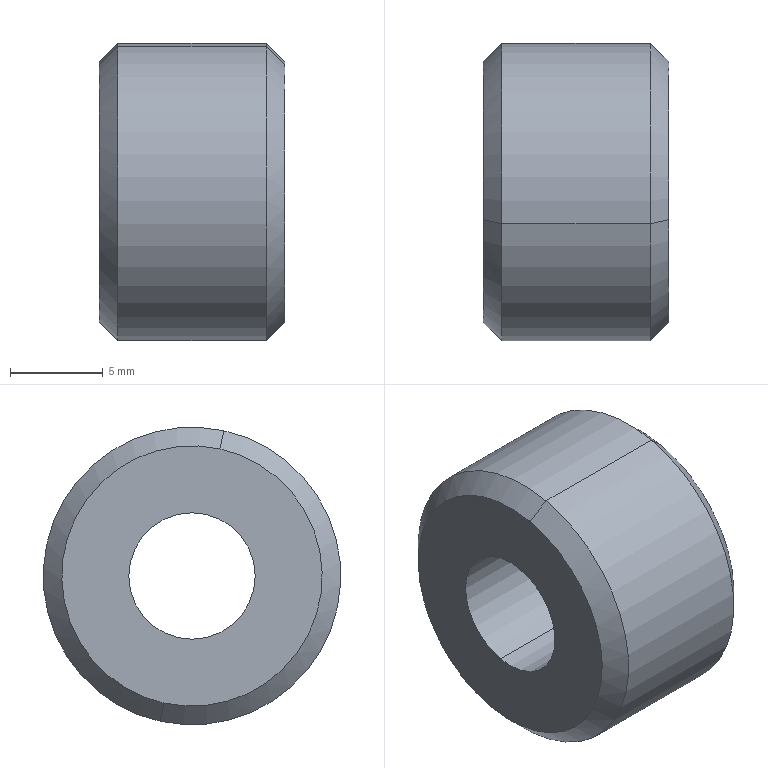Component | SolidWorks | 17SmallKnurledNut-1 | 1 solid | 12 faces | box 10 x 16 x 16 mm | volume 1595 mm3 | cone 6 | cylinder 4 | plane 2 | commonest cylinder face diameters 6.8 x2 16 x2
build123d program:
from build123d import *

# Parameters (mm, degrees)
SKETCH1_R                   = 8
BOSS_EXTRUDE1_DEPTH         = 10
M8_TAPPED_HOLE1_D           = 6.8
M8_TAPPED_HOLE1_DEPTH       = 19.75
M8_TAPPED_HOLE1_CSINK_D     = 8.05
M8_TAPPED_HOLE1_CSINK_ANGLE = 90
M8_TAPPED_HOLE1_TIP         = 2.043
CHAMFER1_SIZE               = 1


with BuildPart() as part:
    # Sketch1 → Boss-Extrude1 (new body)
    with BuildSketch(Plane.XY):
        Circle(SKETCH1_R)
    extrude(amount=BOSS_EXTRUDE1_DEPTH)

    # M8 Tapped Hole1
    with Locations(Plane.XY.offset(10)):
        with Locations((0, 0)):
            CounterSinkHole(M8_TAPPED_HOLE1_D / 2, M8_TAPPED_HOLE1_CSINK_D / 2, depth=M8_TAPPED_HOLE1_DEPTH, counter_sink_angle=M8_TAPPED_HOLE1_CSINK_ANGLE)
            with Locations((0, 0, -(M8_TAPPED_HOLE1_DEPTH + M8_TAPPED_HOLE1_TIP / 2))):  # 118° drill point
                Cone(0, M8_TAPPED_HOLE1_D / 2, M8_TAPPED_HOLE1_TIP, mode=Mode.SUBTRACT)

    # Chamfer1
    chamfer1_edges = [part.edges().sort_by_distance(p)[0] for p in [
        (-8, 0, 0),
        (-8, 0, 10),
    ]]
    chamfer(chamfer1_edges, length=CHAMFER1_SIZE)


solid = part.part

# Placed as in the assembly
solid = solid.moved(Location((-226, 66, -92), (0, 90, 0)))
STEP:
#1=CARTESIAN_POINT('',(-8.504,2.658,-3.891));
#2=VERTEX_POINT('',#1);
#3=CARTESIAN_POINT('',(-8.504,2.539,-3.353));
#4=VERTEX_POINT('',#3);
#5=CARTESIAN_POINT('',(-8.504,2.598,-3.622));
#6=DIRECTION('',(1.,-0.,-0.));
#7=DIRECTION('',(0.,0.2147,-0.9767));
#8=AXIS2_PLACEMENT_3D('',#5,#6,#7);
#9=CIRCLE('',#8,0.2756);
#10=EDGE_CURVE('',#2,#4,#9,.T.);
#11=ORIENTED_EDGE('',*,*,#10,.F.);
#12=CARTESIAN_POINT('',(-8.543,2.666,-3.93));
#13=VERTEX_POINT('',#12);
#14=CARTESIAN_POINT('',(-8.504,2.658,-3.891));
#15=DIRECTION('',(-0.7071,0.1518,-0.6906));
#16=VECTOR('',#15,39.37);
#17=LINE('',#14,#16);
#18=EDGE_CURVE('',#2,#13,#17,.T.);
#19=ORIENTED_EDGE('',*,*,#18,.T.);
#20=CARTESIAN_POINT('',(-8.543,2.531,-3.314));
#21=VERTEX_POINT('',#20);
#22=CARTESIAN_POINT('',(-8.543,2.598,-3.622));
#23=DIRECTION('',(-1.,0.,0.));
#24=DIRECTION('',(0.,0.2147,-0.9767));
#25=AXIS2_PLACEMENT_3D('',#22,#23,#24);
#26=CIRCLE('',#25,0.315);
#27=EDGE_CURVE('',#21,#13,#26,.T.);
#28=ORIENTED_EDGE('',*,*,#27,.F.);
#29=CARTESIAN_POINT('',(-8.504,2.539,-3.353));
#30=DIRECTION('',(-0.7071,-0.1518,0.6906));
#31=VECTOR('',#30,39.37);
#32=LINE('',#29,#31);
#33=EDGE_CURVE('',#4,#21,#32,.T.);
#34=ORIENTED_EDGE('',*,*,#33,.F.);
#35=EDGE_LOOP('',(#11,#19,#28,#34));
#36=FACE_OUTER_BOUND('',#35,.T.);
#37=CARTESIAN_POINT('',(-8.504,2.598,-3.622));
#38=DIRECTION('',(-1.,0.,0.));
#39=DIRECTION('',(0.,-0.2147,0.9767));
#40=AXIS2_PLACEMENT_3D('',#37,#38,#39);
#41=CONICAL_SURFACE('',#40,0.2756,0.7854);
#42=ADVANCED_FACE('',(#36),#41,.T.);
#43=CARTESIAN_POINT('',(-8.898,2.539,-3.353));
#44=VERTEX_POINT('',#43);
#45=CARTESIAN_POINT('',(-8.898,2.658,-3.891));
#46=VERTEX_POINT('',#45);
#47=CARTESIAN_POINT('',(-8.898,2.598,-3.622));
#48=DIRECTION('',(-1.,0.,0.));
#49=DIRECTION('',(0.,0.2147,-0.9767));
#50=AXIS2_PLACEMENT_3D('',#47,#48,#49);
#51=CIRCLE('',#50,0.2756);
#52=EDGE_CURVE('',#44,#46,#51,.T.);
#53=ORIENTED_EDGE('',*,*,#52,.F.);
#54=CARTESIAN_POINT('',(-8.858,2.531,-3.314));
#55=VERTEX_POINT('',#54);
#56=CARTESIAN_POINT('',(-8.858,2.531,-3.314));
#57=DIRECTION('',(0.7071,-0.1518,0.6906));
#58=VECTOR('',#57,39.37);
#59=LINE('',#56,#58);
#60=EDGE_CURVE('',#44,#55,#59,.T.);
#61=ORIENTED_EDGE('',*,*,#60,.T.);
#62=CARTESIAN_POINT('',(-8.858,2.666,-3.93));
#63=VERTEX_POINT('',#62);
#64=CARTESIAN_POINT('',(-8.858,2.598,-3.622));
#65=DIRECTION('',(1.,-0.,-0.));
#66=DIRECTION('',(0.,0.2147,-0.9767));
#67=AXIS2_PLACEMENT_3D('',#64,#65,#66);
#68=CIRCLE('',#67,0.315);
#69=EDGE_CURVE('',#63,#55,#68,.T.);
#70=ORIENTED_EDGE('',*,*,#69,.F.);
#71=CARTESIAN_POINT('',(-8.858,2.666,-3.93));
#72=DIRECTION('',(0.7071,0.1518,-0.6906));
#73=VECTOR('',#72,39.37);
#74=LINE('',#71,#73);
#75=EDGE_CURVE('',#46,#63,#74,.T.);
#76=ORIENTED_EDGE('',*,*,#75,.F.);
#77=EDGE_LOOP('',(#53,#61,#70,#76));
#78=FACE_OUTER_BOUND('',#77,.T.);
#79=CARTESIAN_POINT('',(-8.858,2.598,-3.622));
#80=DIRECTION('',(1.,-0.,-0.));
#81=DIRECTION('',(0.,0.2147,-0.9767));
#82=AXIS2_PLACEMENT_3D('',#79,#80,#81);
#83=CONICAL_SURFACE('',#82,0.315,0.7854);
#84=ADVANCED_FACE('',(#78),#83,.T.);
#85=CARTESIAN_POINT('',(-8.529,2.57,-3.491));
#86=VERTEX_POINT('',#85);
#87=CARTESIAN_POINT('',(-8.529,2.627,-3.753));
#88=VERTEX_POINT('',#87);
#89=CARTESIAN_POINT('',(-8.529,2.598,-3.622));
#90=DIRECTION('',(1.,-0.,-0.));
#91=DIRECTION('',(0.,0.2147,-0.9767));
#92=AXIS2_PLACEMENT_3D('',#89,#90,#91);
#93=CIRCLE('',#92,0.1339);
#94=EDGE_CURVE('',#86,#88,#93,.T.);
#95=ORIENTED_EDGE('',*,*,#94,.F.);
#96=CARTESIAN_POINT('',(-8.504,2.564,-3.467));
#97=VERTEX_POINT('',#96);
#98=CARTESIAN_POINT('',(-8.504,2.564,-3.467));
#99=DIRECTION('',(0.7071,-0.1518,0.6906));
#100=VECTOR('',#99,39.37);
#101=LINE('',#98,#100);
#102=EDGE_CURVE('',#86,#97,#101,.T.);
#103=ORIENTED_EDGE('',*,*,#102,.T.);
#104=CARTESIAN_POINT('',(-8.504,2.632,-3.777));
#105=VERTEX_POINT('',#104);
#106=CARTESIAN_POINT('',(-8.504,2.598,-3.622));
#107=DIRECTION('',(1.,-0.,-0.));
#108=DIRECTION('',(0.,0.2147,-0.9767));
#109=AXIS2_PLACEMENT_3D('',#106,#107,#108);
#110=CIRCLE('',#109,0.1585);
#111=EDGE_CURVE('',#97,#105,#110,.T.);
#112=ORIENTED_EDGE('',*,*,#111,.T.);
#113=CARTESIAN_POINT('',(-8.504,2.632,-3.777));
#114=DIRECTION('',(0.7071,0.1518,-0.6906));
#115=VECTOR('',#114,39.37);
#116=LINE('',#113,#115);
#117=EDGE_CURVE('',#88,#105,#116,.T.);
#118=ORIENTED_EDGE('',*,*,#117,.F.);
#119=EDGE_LOOP('',(#95,#103,#112,#118));
#120=FACE_OUTER_BOUND('',#119,.T.);
#121=CARTESIAN_POINT('',(-8.504,2.598,-3.622));
#122=DIRECTION('',(1.,-0.,-0.));
#123=DIRECTION('',(0.,0.2147,-0.9767));
#124=AXIS2_PLACEMENT_3D('',#121,#122,#123);
#125=CONICAL_SURFACE('',#124,0.1585,0.7854);
#126=ADVANCED_FACE('',(#120),#125,.F.);
#127=CARTESIAN_POINT('',(-8.898,2.57,-3.491));
#128=VERTEX_POINT('',#127);
#129=CARTESIAN_POINT('',(-8.898,2.627,-3.753));
#130=VERTEX_POINT('',#129);
#131=CARTESIAN_POINT('',(-8.898,2.598,-3.622));
#132=DIRECTION('',(1.,-0.,-0.));
#133=DIRECTION('',(0.,0.2147,-0.9767));
#134=AXIS2_PLACEMENT_3D('',#131,#132,#133);
#135=CIRCLE('',#134,0.1339);
#136=EDGE_CURVE('',#128,#130,#135,.T.);
#137=ORIENTED_EDGE('',*,*,#136,.F.);
#138=CARTESIAN_POINT('',(-8.504,2.57,-3.491));
#139=DIRECTION('',(1.,-0.,-0.));
#140=VECTOR('',#139,39.37);
#141=LINE('',#138,#140);
#142=EDGE_CURVE('',#128,#86,#141,.T.);
#143=ORIENTED_EDGE('',*,*,#142,.T.);
#144=ORIENTED_EDGE('',*,*,#94,.T.);
#145=CARTESIAN_POINT('',(-8.504,2.627,-3.753));
#146=DIRECTION('',(1.,-0.,-0.));
#147=VECTOR('',#146,39.37);
#148=LINE('',#145,#147);
#149=EDGE_CURVE('',#130,#88,#148,.T.);
#150=ORIENTED_EDGE('',*,*,#149,.F.);
#151=EDGE_LOOP('',(#137,#143,#144,#150));
#152=FACE_OUTER_BOUND('',#151,.T.);
#153=CARTESIAN_POINT('',(-8.504,2.598,-3.622));
#154=DIRECTION('',(1.,-0.,-0.));
#155=DIRECTION('',(0.,0.2147,-0.9767));
#156=AXIS2_PLACEMENT_3D('',#153,#154,#155);
#157=CYLINDRICAL_SURFACE('',#156,0.1339);
#158=ADVANCED_FACE('',(#152),#157,.F.);
#159=ORIENTED_EDGE('',*,*,#27,.T.);
#160=CARTESIAN_POINT('',(-8.504,2.666,-3.93));
#161=DIRECTION('',(-1.,0.,0.));
#162=VECTOR('',#161,39.37);
#163=LINE('',#160,#162);
#164=EDGE_CURVE('',#13,#63,#163,.T.);
#165=ORIENTED_EDGE('',*,*,#164,.T.);
#166=ORIENTED_EDGE('',*,*,#69,.T.);
#167=CARTESIAN_POINT('',(-8.504,2.531,-3.314));
#168=DIRECTION('',(-1.,0.,0.));
#169=VECTOR('',#168,39.37);
#170=LINE('',#167,#169);
#171=EDGE_CURVE('',#21,#55,#170,.T.);
#172=ORIENTED_EDGE('',*,*,#171,.F.);
#173=EDGE_LOOP('',(#159,#165,#166,#172));
#174=FACE_OUTER_BOUND('',#173,.T.);
#175=CARTESIAN_POINT('',(-8.504,2.598,-3.622));
#176=DIRECTION('',(-1.,0.,0.));
#177=DIRECTION('',(0.,-0.2147,0.9767));
#178=AXIS2_PLACEMENT_3D('',#175,#176,#177);
#179=CYLINDRICAL_SURFACE('',#178,0.315);
#180=ADVANCED_FACE('',(#174),#179,.T.);
#181=ORIENTED_EDGE('',*,*,#164,.F.);
#182=CARTESIAN_POINT('',(-8.543,2.598,-3.622));
#183=DIRECTION('',(-1.,0.,0.));
#184=DIRECTION('',(0.,0.2147,-0.9767));
#185=AXIS2_PLACEMENT_3D('',#182,#183,#184);
#186=CIRCLE('',#185,0.315);
#187=EDGE_CURVE('',#13,#21,#186,.T.);
#188=ORIENTED_EDGE('',*,*,#187,.T.);
#189=ORIENTED_EDGE('',*,*,#171,.T.);
#190=CARTESIAN_POINT('',(-8.858,2.598,-3.622));
#191=DIRECTION('',(1.,-0.,-0.));
#192=DIRECTION('',(0.,0.2147,-0.9767));
#193=AXIS2_PLACEMENT_3D('',#190,#191,#192);
#194=CIRCLE('',#193,0.315);
#195=EDGE_CURVE('',#55,#63,#194,.T.);
#196=ORIENTED_EDGE('',*,*,#195,.T.);
#197=EDGE_LOOP('',(#181,#188,#189,#196));
#198=FACE_OUTER_BOUND('',#197,.T.);
#199=CARTESIAN_POINT('',(-8.504,2.598,-3.622));
#200=DIRECTION('',(-1.,0.,0.));
#201=DIRECTION('',(0.,-0.2147,0.9767));
#202=AXIS2_PLACEMENT_3D('',#199,#200,#201);
#203=CYLINDRICAL_SURFACE('',#202,0.315);
#204=ADVANCED_FACE('',(#198),#203,.T.);
#205=CARTESIAN_POINT('',(-8.504,2.598,-3.622));
#206=DIRECTION('',(1.,-0.,-0.));
#207=DIRECTION('',(0.,0.2147,-0.9767));
#208=AXIS2_PLACEMENT_3D('',#205,#206,#207);
#209=CIRCLE('',#208,0.2756);
#210=EDGE_CURVE('',#4,#2,#209,.T.);
#211=ORIENTED_EDGE('',*,*,#210,.T.);
#212=ORIENTED_EDGE('',*,*,#10,.T.);
#213=EDGE_LOOP('',(#211,#212));
#214=FACE_OUTER_BOUND('',#213,.T.);
#215=CARTESIAN_POINT('',(-8.504,2.598,-3.622));
#216=DIRECTION('',(1.,-0.,-0.));
#217=DIRECTION('',(0.,0.2147,-0.9767));
#218=AXIS2_PLACEMENT_3D('',#215,#216,#217);
#219=CIRCLE('',#218,0.1585);
#220=EDGE_CURVE('',#105,#97,#219,.T.);
#221=ORIENTED_EDGE('',*,*,#220,.F.);
#222=ORIENTED_EDGE('',*,*,#111,.F.);
#223=EDGE_LOOP('',(#221,#222));
#224=FACE_BOUND('',#223,.T.);
#225=CARTESIAN_POINT('',(-8.504,2.598,-3.622));
#226=DIRECTION('',(1.,-0.,-0.));
#227=DIRECTION('',(-0.,0.2147,-0.9767));
#228=AXIS2_PLACEMENT_3D('',#225,#226,#227);
#229=PLANE('',#228);
#230=ADVANCED_FACE('',(#214,#224),#229,.T.);
#231=CARTESIAN_POINT('',(-8.898,2.598,-3.622));
#232=DIRECTION('',(-1.,0.,0.));
#233=DIRECTION('',(0.,0.2147,-0.9767));
#234=AXIS2_PLACEMENT_3D('',#231,#232,#233);
#235=CIRCLE('',#234,0.2756);
#236=EDGE_CURVE('',#46,#44,#235,.T.);
#237=ORIENTED_EDGE('',*,*,#236,.T.);
#238=ORIENTED_EDGE('',*,*,#52,.T.);
#239=EDGE_LOOP('',(#237,#238));
#240=FACE_OUTER_BOUND('',#239,.T.);
#241=CARTESIAN_POINT('',(-8.898,2.598,-3.622));
#242=DIRECTION('',(1.,-0.,-0.));
#243=DIRECTION('',(0.,0.2147,-0.9767));
#244=AXIS2_PLACEMENT_3D('',#241,#242,#243);
#245=CIRCLE('',#244,0.1339);
#246=EDGE_CURVE('',#130,#128,#245,.T.);
#247=ORIENTED_EDGE('',*,*,#246,.T.);
#248=ORIENTED_EDGE('',*,*,#136,.T.);
#249=EDGE_LOOP('',(#247,#248));
#250=FACE_BOUND('',#249,.T.);
#251=CARTESIAN_POINT('',(-8.898,2.598,-3.622));
#252=DIRECTION('',(1.,-0.,-0.));
#253=DIRECTION('',(-0.,0.2147,-0.9767));
#254=AXIS2_PLACEMENT_3D('',#251,#252,#253);
#255=PLANE('',#254);
#256=ADVANCED_FACE('',(#240,#250),#255,.F.);
#257=ORIENTED_EDGE('',*,*,#142,.F.);
#258=ORIENTED_EDGE('',*,*,#246,.F.);
#259=ORIENTED_EDGE('',*,*,#149,.T.);
#260=CARTESIAN_POINT('',(-8.529,2.598,-3.622));
#261=DIRECTION('',(1.,-0.,-0.));
#262=DIRECTION('',(0.,0.2147,-0.9767));
#263=AXIS2_PLACEMENT_3D('',#260,#261,#262);
#264=CIRCLE('',#263,0.1339);
#265=EDGE_CURVE('',#88,#86,#264,.T.);
#266=ORIENTED_EDGE('',*,*,#265,.T.);
#267=EDGE_LOOP('',(#257,#258,#259,#266));
#268=FACE_OUTER_BOUND('',#267,.T.);
#269=CARTESIAN_POINT('',(-8.504,2.598,-3.622));
#270=DIRECTION('',(1.,-0.,-0.));
#271=DIRECTION('',(0.,0.2147,-0.9767));
#272=AXIS2_PLACEMENT_3D('',#269,#270,#271);
#273=CYLINDRICAL_SURFACE('',#272,0.1339);
#274=ADVANCED_FACE('',(#268),#273,.F.);
#275=ORIENTED_EDGE('',*,*,#102,.F.);
#276=ORIENTED_EDGE('',*,*,#265,.F.);
#277=ORIENTED_EDGE('',*,*,#117,.T.);
#278=ORIENTED_EDGE('',*,*,#220,.T.);
#279=EDGE_LOOP('',(#275,#276,#277,#278));
#280=FACE_OUTER_BOUND('',#279,.T.);
#281=CARTESIAN_POINT('',(-8.504,2.598,-3.622));
#282=DIRECTION('',(1.,-0.,-0.));
#283=DIRECTION('',(0.,0.2147,-0.9767));
#284=AXIS2_PLACEMENT_3D('',#281,#282,#283);
#285=CONICAL_SURFACE('',#284,0.1585,0.7854);
#286=ADVANCED_FACE('',(#280),#285,.F.);
#287=ORIENTED_EDGE('',*,*,#60,.F.);
#288=ORIENTED_EDGE('',*,*,#236,.F.);
#289=ORIENTED_EDGE('',*,*,#75,.T.);
#290=ORIENTED_EDGE('',*,*,#195,.F.);
#291=EDGE_LOOP('',(#287,#288,#289,#290));
#292=FACE_OUTER_BOUND('',#291,.T.);
#293=CARTESIAN_POINT('',(-8.858,2.598,-3.622));
#294=DIRECTION('',(1.,-0.,-0.));
#295=DIRECTION('',(0.,0.2147,-0.9767));
#296=AXIS2_PLACEMENT_3D('',#293,#294,#295);
#297=CONICAL_SURFACE('',#296,0.315,0.7854);
#298=ADVANCED_FACE('',(#292),#297,.T.);
#299=ORIENTED_EDGE('',*,*,#18,.F.);
#300=ORIENTED_EDGE('',*,*,#210,.F.);
#301=ORIENTED_EDGE('',*,*,#33,.T.);
#302=ORIENTED_EDGE('',*,*,#187,.F.);
#303=EDGE_LOOP('',(#299,#300,#301,#302));
#304=FACE_OUTER_BOUND('',#303,.T.);
#305=CARTESIAN_POINT('',(-8.504,2.598,-3.622));
#306=DIRECTION('',(-1.,0.,0.));
#307=DIRECTION('',(0.,-0.2147,0.9767));
#308=AXIS2_PLACEMENT_3D('',#305,#306,#307);
#309=CONICAL_SURFACE('',#308,0.2756,0.7854);
#310=ADVANCED_FACE('',(#304),#309,.T.);
#311=CLOSED_SHELL('',(#42,#84,#126,#158,#180,#204,#230,#256,#274,#286,#298,#310));
#312=MANIFOLD_SOLID_BREP('',#311);
#313=CARTESIAN_POINT('',(0.,0.,0.));
#314=DIRECTION('',(0.,0.,1.));
#315=DIRECTION('',(1.,0.,0.));
#316=AXIS2_PLACEMENT_3D('',#313,#314,#315);
#317=(LENGTH_UNIT()NAMED_UNIT(*)SI_UNIT($,.METRE.));
#318=LENGTH_MEASURE_WITH_UNIT(LENGTH_MEASURE(0.0254),#317);
#319=DIMENSIONAL_EXPONENTS(1.,0.,0.,0.,0.,0.,0.);
#320=(CONVERSION_BASED_UNIT('',#318)LENGTH_UNIT()NAMED_UNIT(#319));
#321=UNCERTAINTY_MEASURE_WITH_UNIT(LENGTH_MEASURE(0.00001),#320,'','');
#322=(NAMED_UNIT(*)PLANE_ANGLE_UNIT()SI_UNIT($,.RADIAN.));
#323=(NAMED_UNIT(*)SI_UNIT($,.STERADIAN.)SOLID_ANGLE_UNIT());
#324=(GEOMETRIC_REPRESENTATION_CONTEXT(3)GLOBAL_UNCERTAINTY_ASSIGNED_CONTEXT((#321))GLOBAL_UNIT_ASSIGNED_CONTEXT((#320,#322,#323))REPRESENTATION_CONTEXT('',''));
#325=ADVANCED_BREP_SHAPE_REPRESENTATION('',(#312,#316),#324);
#326=COLOUR_RGB('',0.7922,0.8196,0.9333);
#327=FILL_AREA_STYLE_COLOUR('',#326);
#328=FILL_AREA_STYLE('',(#327));
#329=SURFACE_STYLE_FILL_AREA(#328);
#330=SURFACE_SIDE_STYLE('',(#329));
#331=SURFACE_STYLE_USAGE(.BOTH.,#330);
#332=PRESENTATION_STYLE_ASSIGNMENT((#331));
#333=STYLED_ITEM('',(#332),#312);
#334=PRESENTATION_LAYER_ASSIGNMENT('','',(#333));
#335=(LENGTH_UNIT()NAMED_UNIT(*)SI_UNIT($,.METRE.));
#336=LENGTH_MEASURE_WITH_UNIT(LENGTH_MEASURE(0.0254),#335);
#337=DIMENSIONAL_EXPONENTS(1.,0.,0.,0.,0.,0.,0.);
#338=(CONVERSION_BASED_UNIT('',#336)LENGTH_UNIT()NAMED_UNIT(#337));
#339=UNCERTAINTY_MEASURE_WITH_UNIT(LENGTH_MEASURE(0.00001),#338,'','');
#340=(NAMED_UNIT(*)PLANE_ANGLE_UNIT()SI_UNIT($,.RADIAN.));
#341=(NAMED_UNIT(*)SI_UNIT($,.STERADIAN.)SOLID_ANGLE_UNIT());
#342=(GEOMETRIC_REPRESENTATION_CONTEXT(3)GLOBAL_UNCERTAINTY_ASSIGNED_CONTEXT((#339))GLOBAL_UNIT_ASSIGNED_CONTEXT((#338,#340,#341))REPRESENTATION_CONTEXT('',''));
#343=MECHANICAL_DESIGN_GEOMETRIC_PRESENTATION_REPRESENTATION('',(#333),#342);